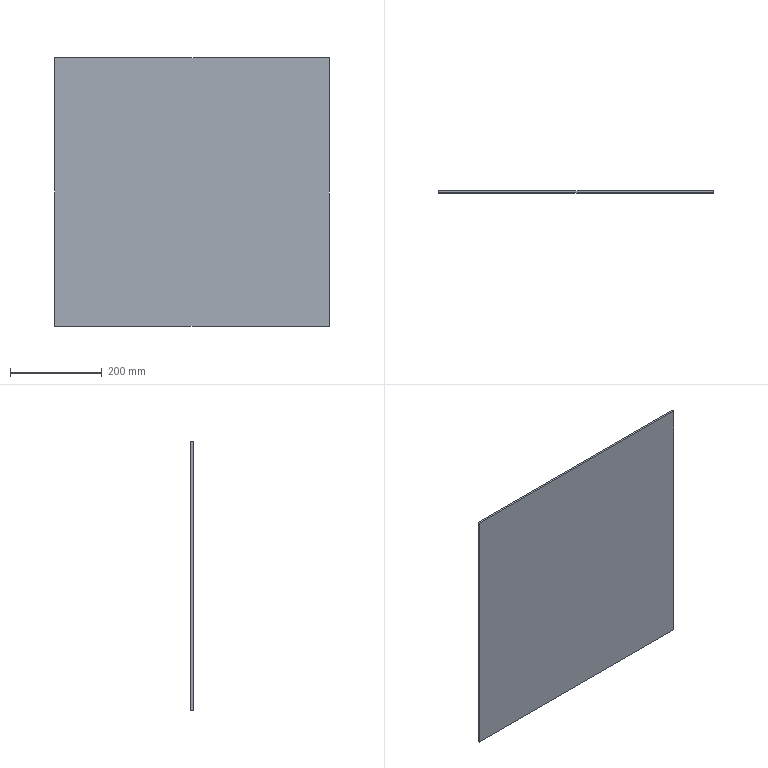Component | SolidWorks | CoverPlate4-1 | 1 solid | 6 faces | box 600 x 5 x 585 mm | volume 1755000 mm3 | plane 6
build123d program:
from build123d import *

# Parameters (mm, degrees)
SKETCH1_W      = 600
SKETCH1_H      = 585
EXTRUDE1_DEPTH = 5


with BuildPart() as part:
    # Sketch1 → Extrude1 (new body)
    with BuildSketch(Plane.XY):
        Rectangle(SKETCH1_W, SKETCH1_H)
    extrude(amount=EXTRUDE1_DEPTH)


solid = part.part

# Placed as in the assembly
solid = solid.moved(Location((15, 615, 272.5), (90, 0, 0)))
STEP:
#1=COLOUR_RGB('',0.7922,0.8196,0.9333);
#2=FILL_AREA_STYLE_COLOUR('',#1);
#3=FILL_AREA_STYLE('',(#2));
#4=SURFACE_STYLE_FILL_AREA(#3);
#5=SURFACE_SIDE_STYLE('',(#4));
#6=SURFACE_STYLE_USAGE(.BOTH.,#5);
#7=PRESENTATION_STYLE_ASSIGNMENT((#6));
#8=CARTESIAN_POINT('',(12.402,24.016,22.244));
#9=VERTEX_POINT('',#8);
#10=CARTESIAN_POINT('',(12.402,24.016,-0.7874));
#11=VERTEX_POINT('',#10);
#12=CARTESIAN_POINT('',(12.402,24.016,-0.7874));
#13=DIRECTION('',(0.,0.,-1.));
#14=VECTOR('',#13,39.37);
#15=LINE('',#12,#14);
#16=EDGE_CURVE('',#9,#11,#15,.T.);
#17=ORIENTED_EDGE('',*,*,#16,.T.);
#18=CARTESIAN_POINT('',(12.402,24.213,-0.7874));
#19=VERTEX_POINT('',#18);
#20=CARTESIAN_POINT('',(12.402,24.213,-0.7874));
#21=DIRECTION('',(-0.,-1.,-0.));
#22=VECTOR('',#21,39.37);
#23=LINE('',#20,#22);
#24=EDGE_CURVE('',#19,#11,#23,.T.);
#25=ORIENTED_EDGE('',*,*,#24,.F.);
#26=CARTESIAN_POINT('',(12.402,24.213,22.244));
#27=VERTEX_POINT('',#26);
#28=CARTESIAN_POINT('',(12.402,24.213,-0.7874));
#29=DIRECTION('',(0.,0.,-1.));
#30=VECTOR('',#29,39.37);
#31=LINE('',#28,#30);
#32=EDGE_CURVE('',#27,#19,#31,.T.);
#33=ORIENTED_EDGE('',*,*,#32,.F.);
#34=CARTESIAN_POINT('',(12.402,24.213,22.244));
#35=DIRECTION('',(-0.,-1.,-0.));
#36=VECTOR('',#35,39.37);
#37=LINE('',#34,#36);
#38=EDGE_CURVE('',#27,#9,#37,.T.);
#39=ORIENTED_EDGE('',*,*,#38,.T.);
#40=EDGE_LOOP('',(#17,#25,#33,#39));
#41=FACE_OUTER_BOUND('',#40,.T.);
#42=CARTESIAN_POINT('',(12.402,24.213,-0.7874));
#43=DIRECTION('',(-1.,0.,-0.));
#44=DIRECTION('',(-0.,-0.,1.));
#45=AXIS2_PLACEMENT_3D('',#42,#43,#44);
#46=PLANE('',#45);
#47=ADVANCED_FACE('',(#41),#46,.F.);
#48=CARTESIAN_POINT('',(-11.22,24.016,-0.7874));
#49=VERTEX_POINT('',#48);
#50=CARTESIAN_POINT('',(-11.22,24.016,-0.7874));
#51=DIRECTION('',(-1.,0.,-0.));
#52=VECTOR('',#51,39.37);
#53=LINE('',#50,#52);
#54=EDGE_CURVE('',#11,#49,#53,.T.);
#55=ORIENTED_EDGE('',*,*,#54,.T.);
#56=CARTESIAN_POINT('',(-11.22,24.213,-0.7874));
#57=VERTEX_POINT('',#56);
#58=CARTESIAN_POINT('',(-11.22,24.213,-0.7874));
#59=DIRECTION('',(-0.,-1.,-0.));
#60=VECTOR('',#59,39.37);
#61=LINE('',#58,#60);
#62=EDGE_CURVE('',#57,#49,#61,.T.);
#63=ORIENTED_EDGE('',*,*,#62,.F.);
#64=CARTESIAN_POINT('',(-11.22,24.213,-0.7874));
#65=DIRECTION('',(-1.,0.,-0.));
#66=VECTOR('',#65,39.37);
#67=LINE('',#64,#66);
#68=EDGE_CURVE('',#19,#57,#67,.T.);
#69=ORIENTED_EDGE('',*,*,#68,.F.);
#70=ORIENTED_EDGE('',*,*,#24,.T.);
#71=EDGE_LOOP('',(#55,#63,#69,#70));
#72=FACE_OUTER_BOUND('',#71,.T.);
#73=CARTESIAN_POINT('',(-11.22,24.213,-0.7874));
#74=DIRECTION('',(-0.,-0.,1.));
#75=DIRECTION('',(-0.,-1.,-0.));
#76=AXIS2_PLACEMENT_3D('',#73,#74,#75);
#77=PLANE('',#76);
#78=ADVANCED_FACE('',(#72),#77,.F.);
#79=CARTESIAN_POINT('',(-11.22,24.016,22.244));
#80=VERTEX_POINT('',#79);
#81=CARTESIAN_POINT('',(-11.22,24.016,-0.7874));
#82=DIRECTION('',(-0.,-0.,1.));
#83=VECTOR('',#82,39.37);
#84=LINE('',#81,#83);
#85=EDGE_CURVE('',#49,#80,#84,.T.);
#86=ORIENTED_EDGE('',*,*,#85,.T.);
#87=CARTESIAN_POINT('',(-11.22,24.213,22.244));
#88=VERTEX_POINT('',#87);
#89=CARTESIAN_POINT('',(-11.22,24.213,22.244));
#90=DIRECTION('',(-0.,-1.,-0.));
#91=VECTOR('',#90,39.37);
#92=LINE('',#89,#91);
#93=EDGE_CURVE('',#88,#80,#92,.T.);
#94=ORIENTED_EDGE('',*,*,#93,.F.);
#95=CARTESIAN_POINT('',(-11.22,24.213,-0.7874));
#96=DIRECTION('',(-0.,-0.,1.));
#97=VECTOR('',#96,39.37);
#98=LINE('',#95,#97);
#99=EDGE_CURVE('',#57,#88,#98,.T.);
#100=ORIENTED_EDGE('',*,*,#99,.F.);
#101=ORIENTED_EDGE('',*,*,#62,.T.);
#102=EDGE_LOOP('',(#86,#94,#100,#101));
#103=FACE_OUTER_BOUND('',#102,.T.);
#104=CARTESIAN_POINT('',(-11.22,24.213,-0.7874));
#105=DIRECTION('',(1.,-0.,0.));
#106=DIRECTION('',(0.,0.,-1.));
#107=AXIS2_PLACEMENT_3D('',#104,#105,#106);
#108=PLANE('',#107);
#109=ADVANCED_FACE('',(#103),#108,.F.);
#110=CARTESIAN_POINT('',(-11.22,24.016,22.244));
#111=DIRECTION('',(1.,-0.,0.));
#112=VECTOR('',#111,39.37);
#113=LINE('',#110,#112);
#114=EDGE_CURVE('',#80,#9,#113,.T.);
#115=ORIENTED_EDGE('',*,*,#114,.T.);
#116=ORIENTED_EDGE('',*,*,#38,.F.);
#117=CARTESIAN_POINT('',(-11.22,24.213,22.244));
#118=DIRECTION('',(1.,-0.,0.));
#119=VECTOR('',#118,39.37);
#120=LINE('',#117,#119);
#121=EDGE_CURVE('',#88,#27,#120,.T.);
#122=ORIENTED_EDGE('',*,*,#121,.F.);
#123=ORIENTED_EDGE('',*,*,#93,.T.);
#124=EDGE_LOOP('',(#115,#116,#122,#123));
#125=FACE_OUTER_BOUND('',#124,.T.);
#126=CARTESIAN_POINT('',(-11.22,24.213,22.244));
#127=DIRECTION('',(0.,0.,-1.));
#128=DIRECTION('',(0.,1.,0.));
#129=AXIS2_PLACEMENT_3D('',#126,#127,#128);
#130=PLANE('',#129);
#131=ADVANCED_FACE('',(#125),#130,.F.);
#132=ORIENTED_EDGE('',*,*,#32,.T.);
#133=ORIENTED_EDGE('',*,*,#68,.T.);
#134=ORIENTED_EDGE('',*,*,#99,.T.);
#135=ORIENTED_EDGE('',*,*,#121,.T.);
#136=EDGE_LOOP('',(#132,#133,#134,#135));
#137=FACE_OUTER_BOUND('',#136,.T.);
#138=CARTESIAN_POINT('',(0.5906,24.213,10.728));
#139=DIRECTION('',(0.,1.,0.));
#140=DIRECTION('',(1.,-0.,0.));
#141=AXIS2_PLACEMENT_3D('',#138,#139,#140);
#142=PLANE('',#141);
#143=ADVANCED_FACE('',(#137),#142,.T.);
#144=ORIENTED_EDGE('',*,*,#16,.F.);
#145=ORIENTED_EDGE('',*,*,#114,.F.);
#146=ORIENTED_EDGE('',*,*,#85,.F.);
#147=ORIENTED_EDGE('',*,*,#54,.F.);
#148=EDGE_LOOP('',(#144,#145,#146,#147));
#149=FACE_OUTER_BOUND('',#148,.T.);
#150=CARTESIAN_POINT('',(0.5906,24.016,10.728));
#151=DIRECTION('',(0.,1.,0.));
#152=DIRECTION('',(1.,-0.,0.));
#153=AXIS2_PLACEMENT_3D('',#150,#151,#152);
#154=PLANE('',#153);
#155=ADVANCED_FACE('',(#149),#154,.F.);
#156=CLOSED_SHELL('',(#47,#78,#109,#131,#143,#155));
#157=MANIFOLD_SOLID_BREP('',#156);
#158=STYLED_ITEM('',(#7),#157);
#159=(LENGTH_UNIT()NAMED_UNIT(*)SI_UNIT($,.METRE.));
#160=LENGTH_MEASURE_WITH_UNIT(LENGTH_MEASURE(0.0254),#159);
#161=DIMENSIONAL_EXPONENTS(1.,0.,0.,0.,0.,0.,0.);
#162=(CONVERSION_BASED_UNIT('',#160)LENGTH_UNIT()NAMED_UNIT(#161));
#163=UNCERTAINTY_MEASURE_WITH_UNIT(LENGTH_MEASURE(0.00001),#162,'','');
#164=(NAMED_UNIT(*)PLANE_ANGLE_UNIT()SI_UNIT($,.RADIAN.));
#165=(NAMED_UNIT(*)SI_UNIT($,.STERADIAN.)SOLID_ANGLE_UNIT());
#166=(GEOMETRIC_REPRESENTATION_CONTEXT(3)GLOBAL_UNCERTAINTY_ASSIGNED_CONTEXT((#163))GLOBAL_UNIT_ASSIGNED_CONTEXT((#162,#164,#165))REPRESENTATION_CONTEXT('',''));
#167=MECHANICAL_DESIGN_GEOMETRIC_PRESENTATION_REPRESENTATION('',(#158),#166);
#168=CARTESIAN_POINT('',(0.,0.,0.));
#169=DIRECTION('',(0.,0.,1.));
#170=DIRECTION('',(1.,0.,0.));
#171=AXIS2_PLACEMENT_3D('',#168,#169,#170);
#172=(LENGTH_UNIT()NAMED_UNIT(*)SI_UNIT($,.METRE.));
#173=LENGTH_MEASURE_WITH_UNIT(LENGTH_MEASURE(0.0254),#172);
#174=DIMENSIONAL_EXPONENTS(1.,0.,0.,0.,0.,0.,0.);
#175=(CONVERSION_BASED_UNIT('',#173)LENGTH_UNIT()NAMED_UNIT(#174));
#176=UNCERTAINTY_MEASURE_WITH_UNIT(LENGTH_MEASURE(0.00001),#175,'','');
#177=(NAMED_UNIT(*)PLANE_ANGLE_UNIT()SI_UNIT($,.RADIAN.));
#178=(NAMED_UNIT(*)SI_UNIT($,.STERADIAN.)SOLID_ANGLE_UNIT());
#179=(GEOMETRIC_REPRESENTATION_CONTEXT(3)GLOBAL_UNCERTAINTY_ASSIGNED_CONTEXT((#176))GLOBAL_UNIT_ASSIGNED_CONTEXT((#175,#177,#178))REPRESENTATION_CONTEXT('',''));
#180=ADVANCED_BREP_SHAPE_REPRESENTATION('',(#157,#171),#179);
#181=PRESENTATION_LAYER_ASSIGNMENT('','',(#158));